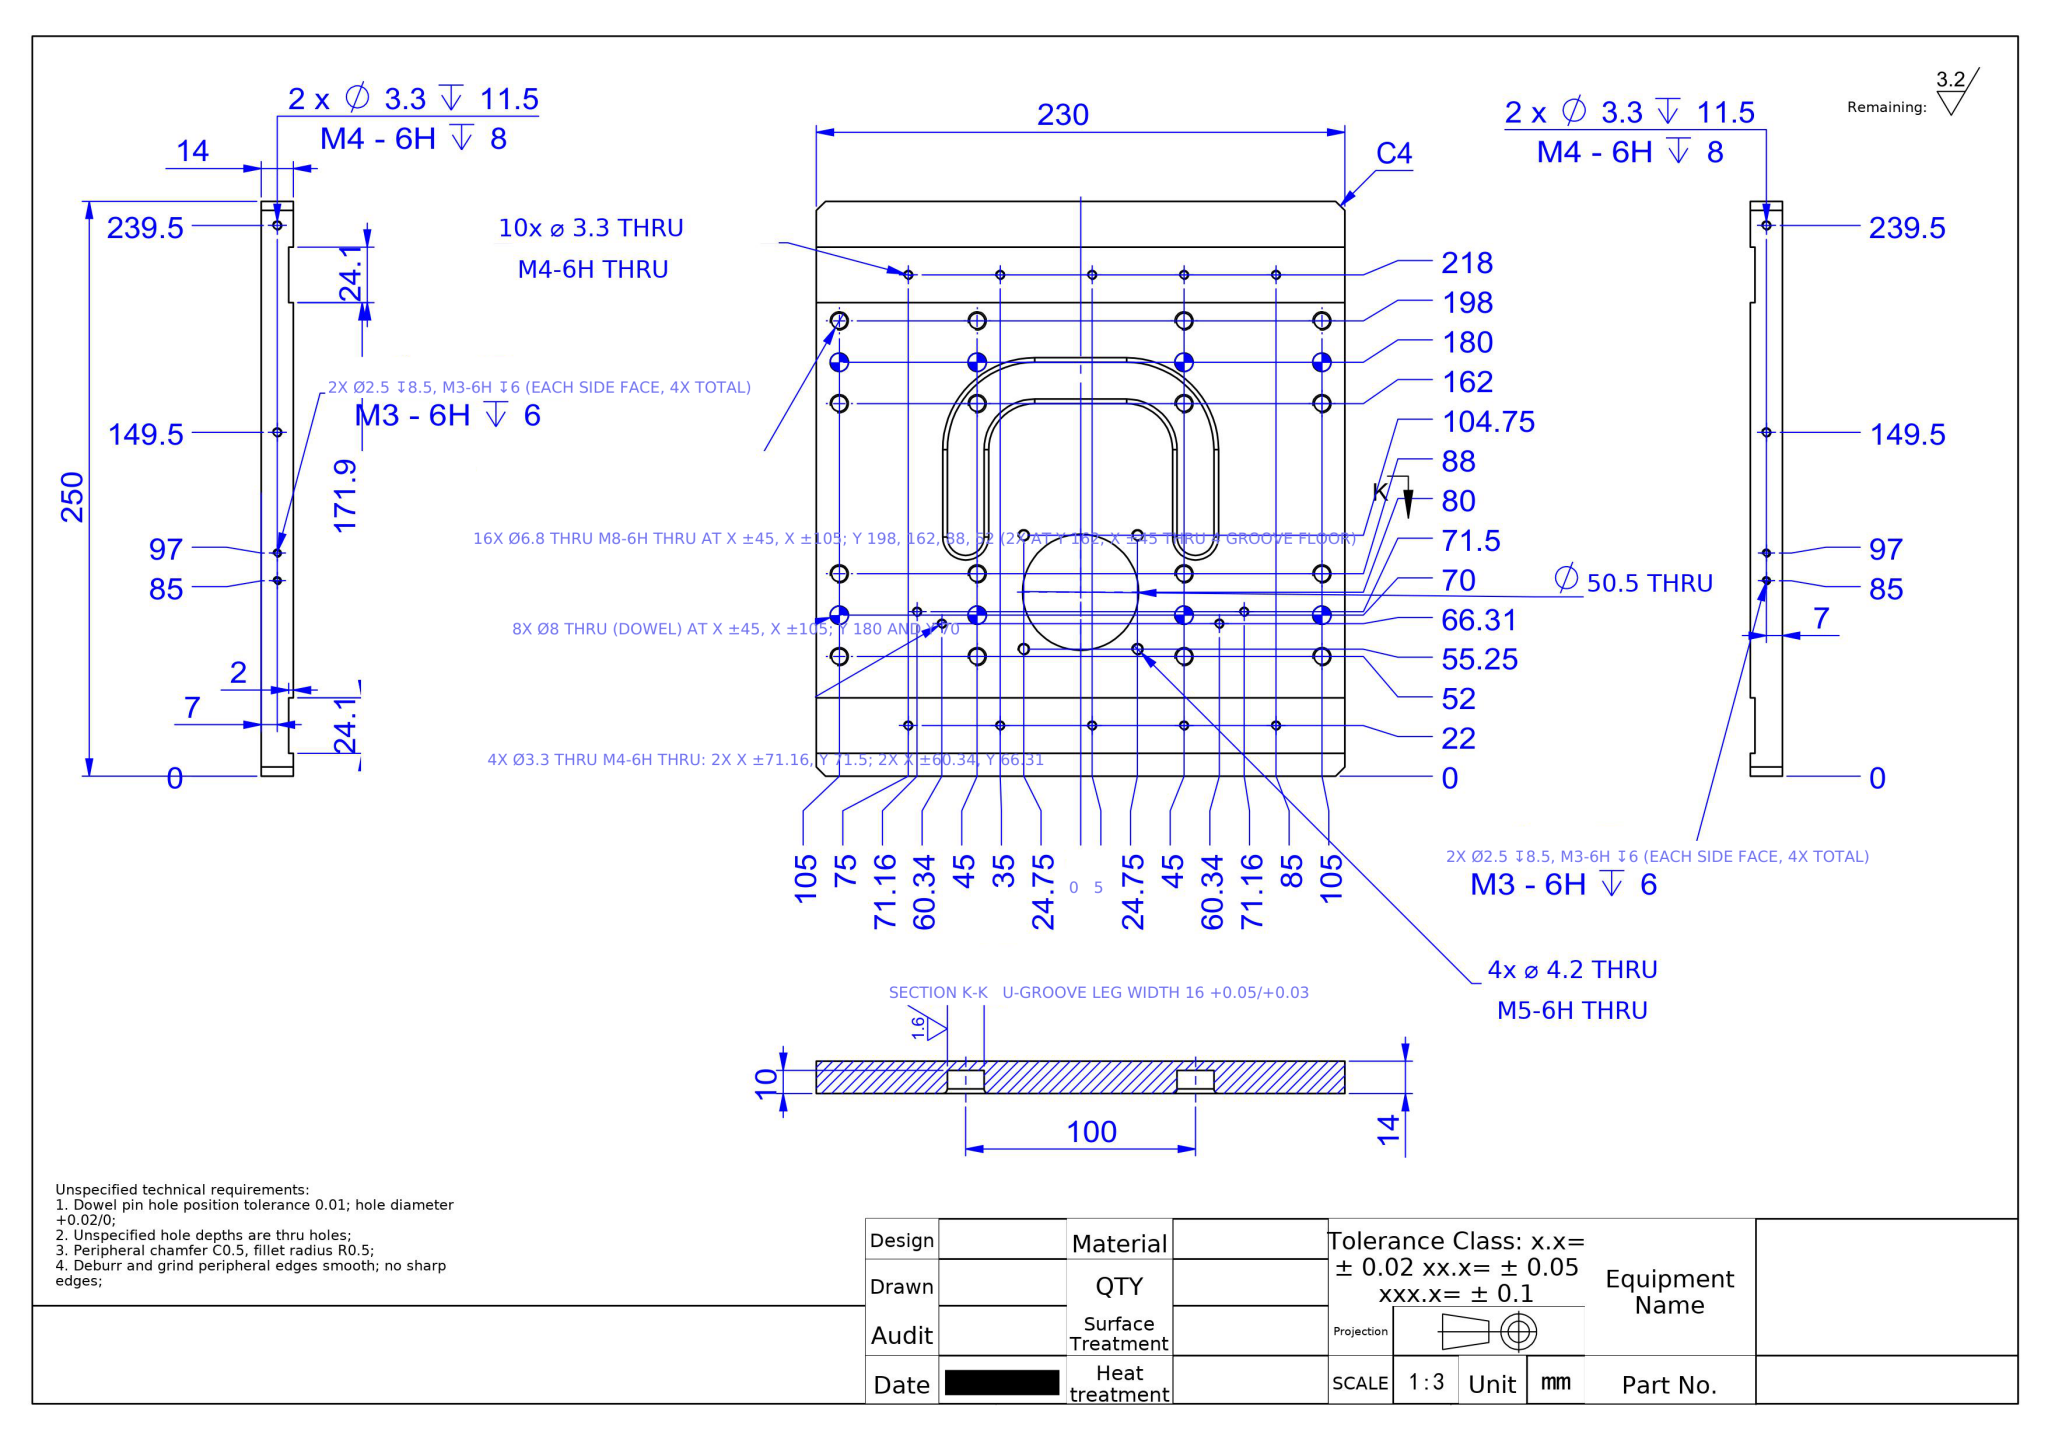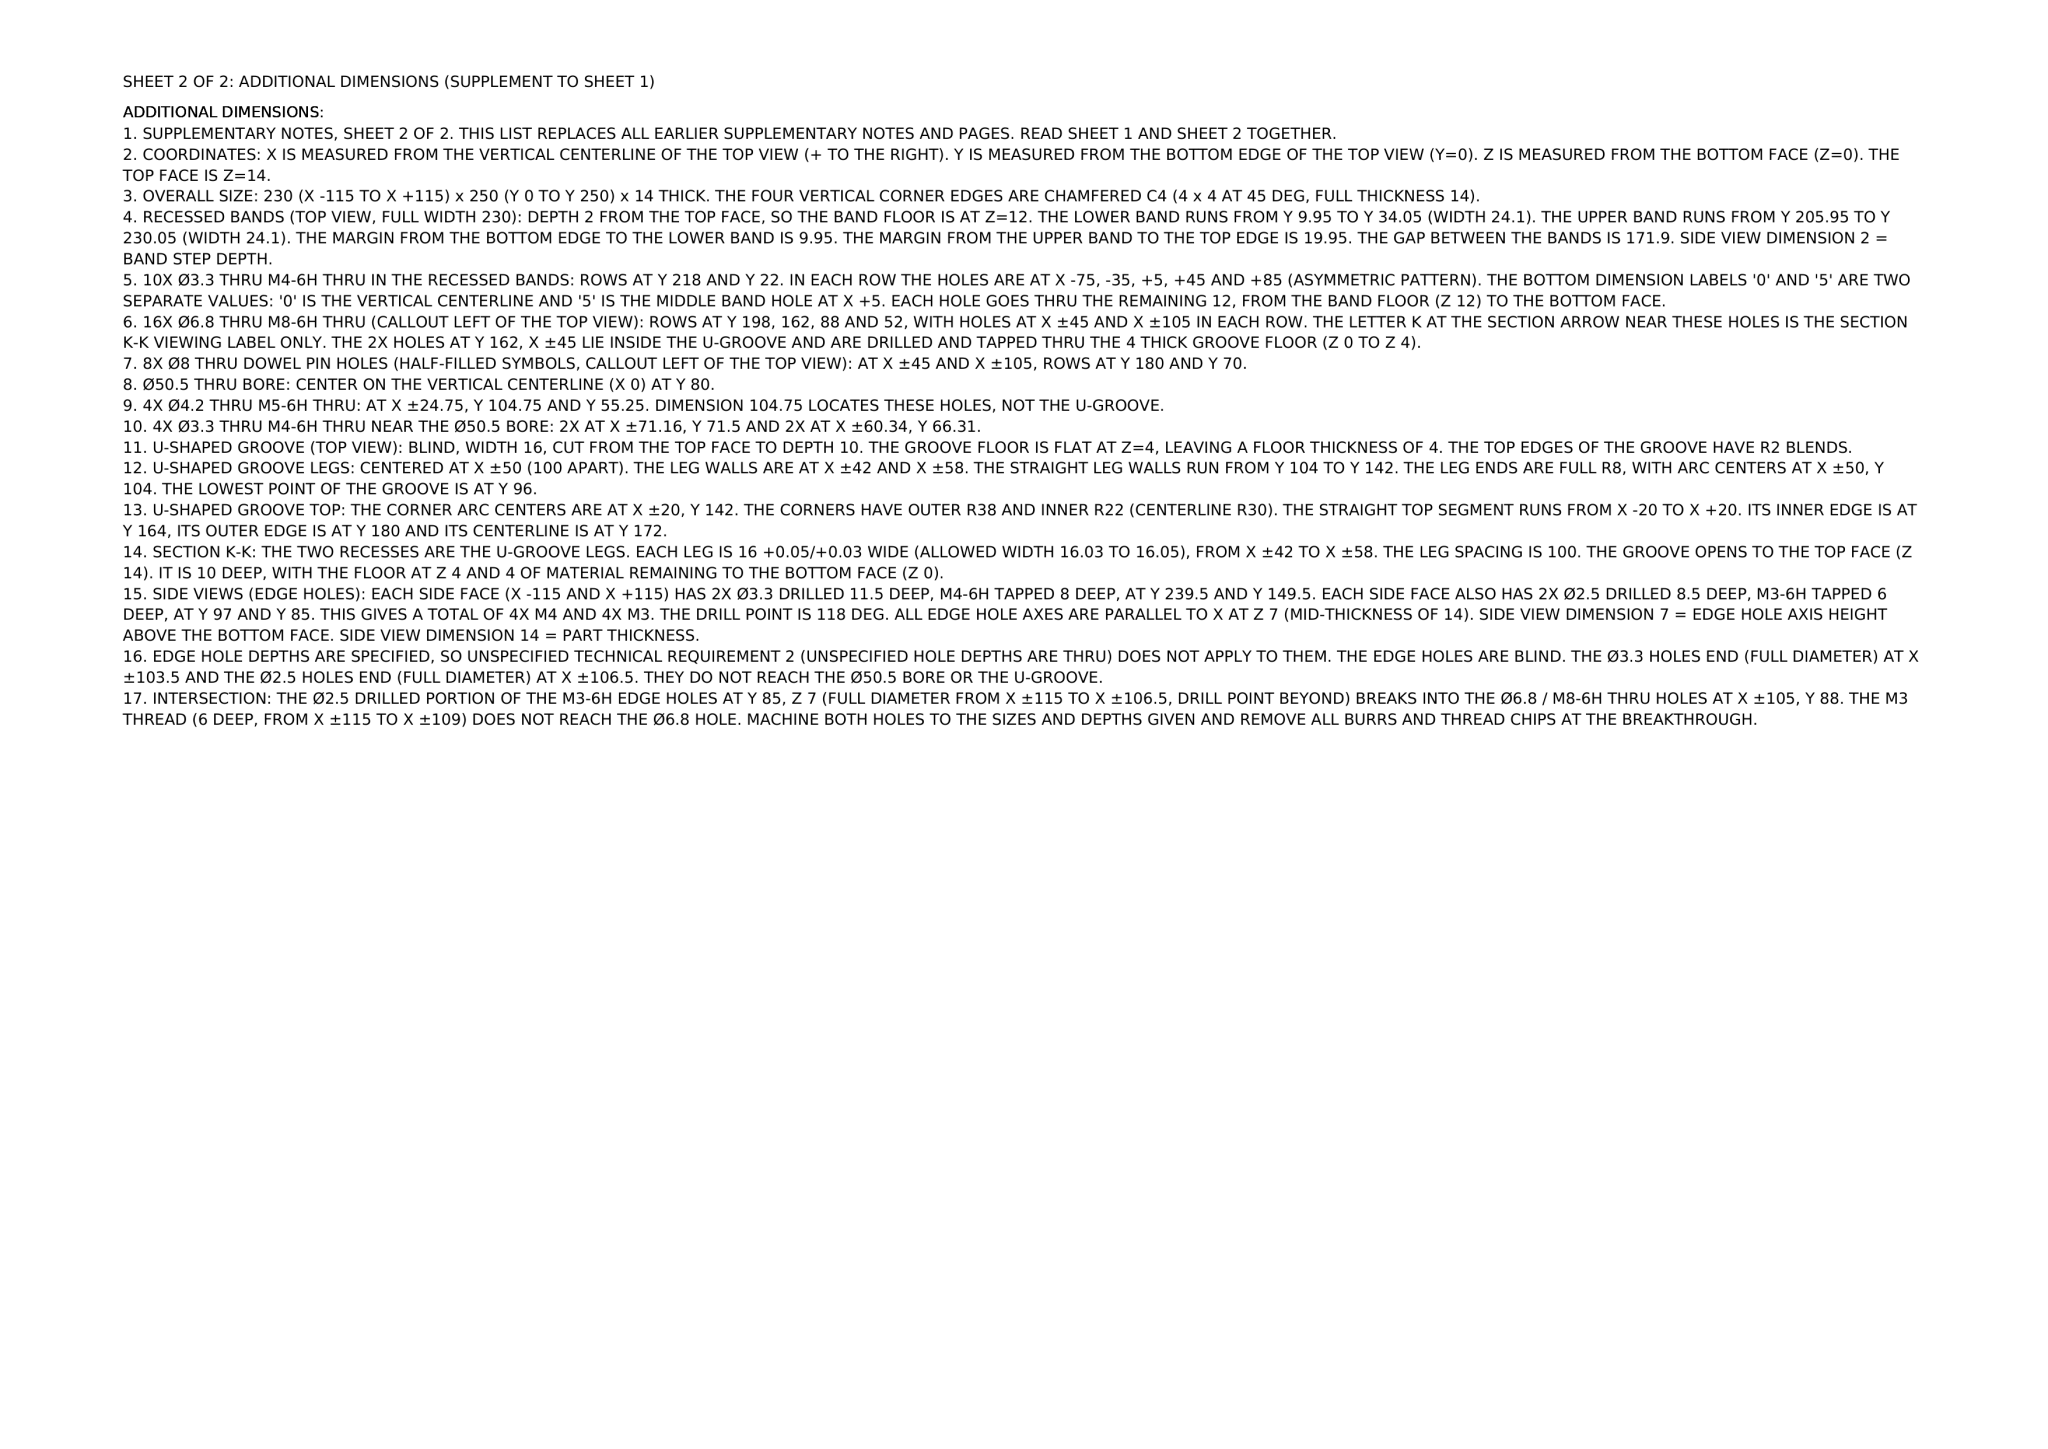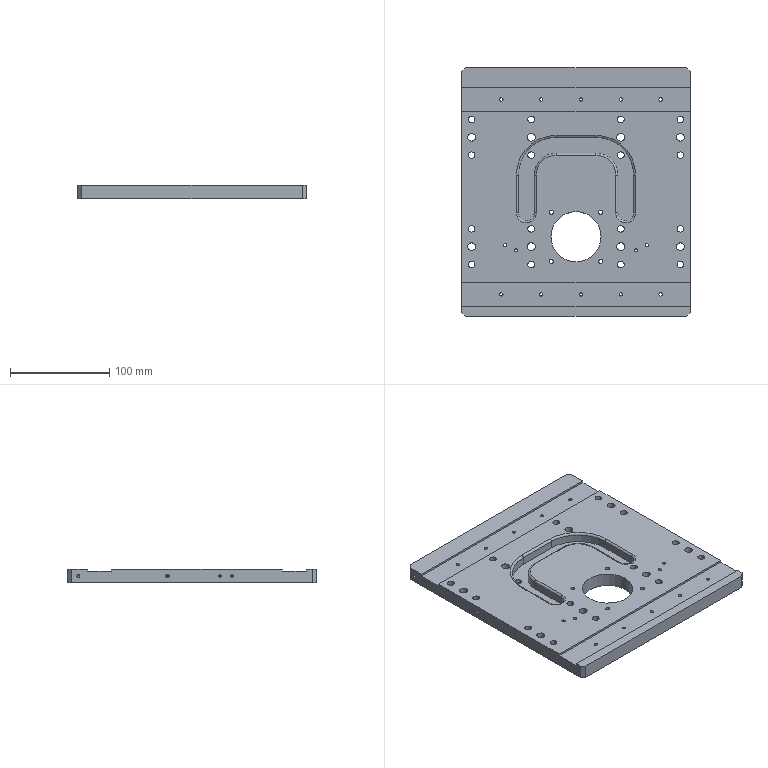Part | NX | mm | 1 solid | 159 faces | box 230 x 250 x 14 mm | volume 702391 mm3 | cylinder 114 | plane 25 | cone 14 | torus 6 | commonest cylinder face diameters 3.3 x36 6.8 x32 8 x16 4.2 x8 2.5 x8 4 x6 50.5 x2 16 x2